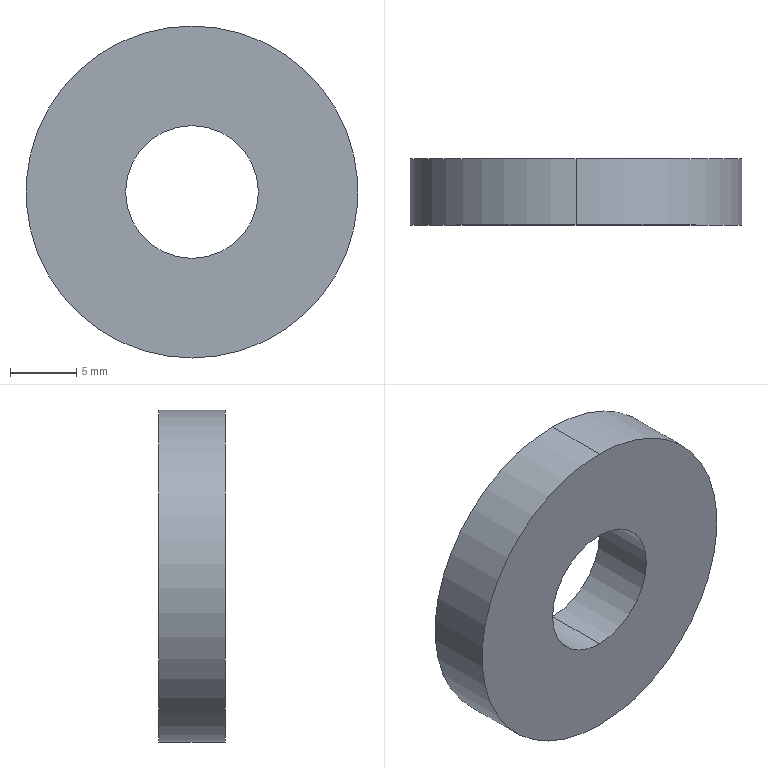Component | SolidWorks | STB-08-022-1 | 1 solid | 6 faces | box 25 x 5 x 25 mm | volume 2062 mm3 | cylinder 4 | plane 2 | commonest cylinder face diameters 10 x2 25 x2
build123d program:
from build123d import *

# Parameters (mm, degrees)
SKETCH1_R           = 12.5
BOSS_EXTRUDE1_DEPTH = 2.5
CUT_EXTRUDE1_REACH  = 20.371
SKETCH2_R           = 5


with BuildPart() as part:
    # Sketch1 → Boss-Extrude1 (new, symmetric)
    with BuildSketch(Plane(origin=(0, 0, 0), x_dir=(1, 0, 0), z_dir=(0, 1, 0))):
        with Locations(Location((0, 0, 0), (0, 0, 270))):
            Circle(SKETCH1_R)
    extrude(amount=BOSS_EXTRUDE1_DEPTH, both=True)

    # Sketch2 → Cut-Extrude1 (cut, up to next)
    with BuildSketch(Plane(origin=(0, 2.5, 0), x_dir=(1, 0, 0), z_dir=(0, 1, 0)), mode=Mode.PRIVATE) as cut_extrude1_sk1:
        with Locations(Location((0, 0, 0), (0, 0, 270))):
            Circle(SKETCH2_R)
    cut_extrude1_tool1 = extrude(cut_extrude1_sk1.sketch, amount=-CUT_EXTRUDE1_REACH, mode=Mode.PRIVATE) & part.part
    add(cut_extrude1_tool1.solids().sort_by_distance((0, 2.5, 0))[0], mode=Mode.SUBTRACT)


solid = part.part

# Placed as in the assembly
solid = solid.moved(Location((-149.904, 246.499, -12), (0, 0, 0)))
STEP:
#1=COLOUR_RGB('',0.7922,0.8196,0.9333);
#2=FILL_AREA_STYLE_COLOUR('',#1);
#3=FILL_AREA_STYLE('',(#2));
#4=SURFACE_STYLE_FILL_AREA(#3);
#5=SURFACE_SIDE_STYLE('',(#4));
#6=SURFACE_STYLE_USAGE(.BOTH.,#5);
#7=PRESENTATION_STYLE_ASSIGNMENT((#6));
#8=CARTESIAN_POINT('',(-5.902,9.606,-0.2756));
#9=VERTEX_POINT('',#8);
#10=CARTESIAN_POINT('',(-5.902,9.606,-0.6693));
#11=VERTEX_POINT('',#10);
#12=CARTESIAN_POINT('',(-5.902,9.606,-0.4724));
#13=DIRECTION('',(0.,-1.,0.));
#14=DIRECTION('',(0.,0.,1.));
#15=AXIS2_PLACEMENT_3D('',#12,#13,#14);
#16=CIRCLE('',#15,0.1969);
#17=EDGE_CURVE('',#9,#11,#16,.T.);
#18=ORIENTED_EDGE('',*,*,#17,.T.);
#19=CARTESIAN_POINT('',(-5.902,9.803,-0.6693));
#20=VERTEX_POINT('',#19);
#21=CARTESIAN_POINT('',(-5.902,9.606,-0.6693));
#22=DIRECTION('',(0.,1.,0.));
#23=VECTOR('',#22,39.37);
#24=LINE('',#21,#23);
#25=EDGE_CURVE('',#11,#20,#24,.T.);
#26=ORIENTED_EDGE('',*,*,#25,.T.);
#27=CARTESIAN_POINT('',(-5.902,9.803,-0.2756));
#28=VERTEX_POINT('',#27);
#29=CARTESIAN_POINT('',(-5.902,9.803,-0.4724));
#30=DIRECTION('',(0.,1.,0.));
#31=DIRECTION('',(0.,0.,1.));
#32=AXIS2_PLACEMENT_3D('',#29,#30,#31);
#33=CIRCLE('',#32,0.1969);
#34=EDGE_CURVE('',#20,#28,#33,.T.);
#35=ORIENTED_EDGE('',*,*,#34,.T.);
#36=CARTESIAN_POINT('',(-5.902,9.606,-0.2756));
#37=DIRECTION('',(0.,1.,0.));
#38=VECTOR('',#37,39.37);
#39=LINE('',#36,#38);
#40=EDGE_CURVE('',#9,#28,#39,.T.);
#41=ORIENTED_EDGE('',*,*,#40,.F.);
#42=EDGE_LOOP('',(#18,#26,#35,#41));
#43=FACE_OUTER_BOUND('',#42,.T.);
#44=CARTESIAN_POINT('',(-5.902,9.606,-0.4724));
#45=DIRECTION('',(0.,1.,0.));
#46=DIRECTION('',(0.,0.,1.));
#47=AXIS2_PLACEMENT_3D('',#44,#45,#46);
#48=CYLINDRICAL_SURFACE('',#47,0.1969);
#49=ADVANCED_FACE('',(#43),#48,.F.);
#50=CARTESIAN_POINT('',(-5.902,9.803,0.01969));
#51=VERTEX_POINT('',#50);
#52=CARTESIAN_POINT('',(-5.902,9.803,-0.9646));
#53=VERTEX_POINT('',#52);
#54=CARTESIAN_POINT('',(-5.902,9.803,-0.4724));
#55=DIRECTION('',(0.,1.,0.));
#56=DIRECTION('',(0.,0.,1.));
#57=AXIS2_PLACEMENT_3D('',#54,#55,#56);
#58=CIRCLE('',#57,0.4921);
#59=EDGE_CURVE('',#51,#53,#58,.T.);
#60=ORIENTED_EDGE('',*,*,#59,.F.);
#61=CARTESIAN_POINT('',(-5.902,9.606,0.01969));
#62=VERTEX_POINT('',#61);
#63=CARTESIAN_POINT('',(-5.902,9.803,0.01969));
#64=DIRECTION('',(0.,-1.,0.));
#65=VECTOR('',#64,39.37);
#66=LINE('',#63,#65);
#67=EDGE_CURVE('',#51,#62,#66,.T.);
#68=ORIENTED_EDGE('',*,*,#67,.T.);
#69=CARTESIAN_POINT('',(-5.902,9.606,-0.9646));
#70=VERTEX_POINT('',#69);
#71=CARTESIAN_POINT('',(-5.902,9.606,-0.4724));
#72=DIRECTION('',(0.,1.,0.));
#73=DIRECTION('',(0.,0.,1.));
#74=AXIS2_PLACEMENT_3D('',#71,#72,#73);
#75=CIRCLE('',#74,0.4921);
#76=EDGE_CURVE('',#62,#70,#75,.T.);
#77=ORIENTED_EDGE('',*,*,#76,.T.);
#78=CARTESIAN_POINT('',(-5.902,9.803,-0.9646));
#79=DIRECTION('',(0.,-1.,0.));
#80=VECTOR('',#79,39.37);
#81=LINE('',#78,#80);
#82=EDGE_CURVE('',#53,#70,#81,.T.);
#83=ORIENTED_EDGE('',*,*,#82,.F.);
#84=EDGE_LOOP('',(#60,#68,#77,#83));
#85=FACE_OUTER_BOUND('',#84,.T.);
#86=CARTESIAN_POINT('',(-5.902,9.803,-0.4724));
#87=DIRECTION('',(0.,-1.,0.));
#88=DIRECTION('',(0.,0.,-1.));
#89=AXIS2_PLACEMENT_3D('',#86,#87,#88);
#90=CYLINDRICAL_SURFACE('',#89,0.4921);
#91=ADVANCED_FACE('',(#85),#90,.T.);
#92=ORIENTED_EDGE('',*,*,#67,.F.);
#93=CARTESIAN_POINT('',(-5.902,9.803,-0.4724));
#94=DIRECTION('',(0.,1.,0.));
#95=DIRECTION('',(0.,0.,1.));
#96=AXIS2_PLACEMENT_3D('',#93,#94,#95);
#97=CIRCLE('',#96,0.4921);
#98=EDGE_CURVE('',#53,#51,#97,.T.);
#99=ORIENTED_EDGE('',*,*,#98,.F.);
#100=ORIENTED_EDGE('',*,*,#82,.T.);
#101=CARTESIAN_POINT('',(-5.902,9.606,-0.4724));
#102=DIRECTION('',(0.,1.,0.));
#103=DIRECTION('',(0.,0.,1.));
#104=AXIS2_PLACEMENT_3D('',#101,#102,#103);
#105=CIRCLE('',#104,0.4921);
#106=EDGE_CURVE('',#70,#62,#105,.T.);
#107=ORIENTED_EDGE('',*,*,#106,.T.);
#108=EDGE_LOOP('',(#92,#99,#100,#107));
#109=FACE_OUTER_BOUND('',#108,.T.);
#110=CARTESIAN_POINT('',(-5.902,9.803,-0.4724));
#111=DIRECTION('',(0.,-1.,0.));
#112=DIRECTION('',(0.,0.,-1.));
#113=AXIS2_PLACEMENT_3D('',#110,#111,#112);
#114=CYLINDRICAL_SURFACE('',#113,0.4921);
#115=ADVANCED_FACE('',(#109),#114,.T.);
#116=CARTESIAN_POINT('',(-5.902,9.803,-0.4724));
#117=DIRECTION('',(0.,1.,0.));
#118=DIRECTION('',(0.,0.,1.));
#119=AXIS2_PLACEMENT_3D('',#116,#117,#118);
#120=CIRCLE('',#119,0.1969);
#121=EDGE_CURVE('',#28,#20,#120,.T.);
#122=ORIENTED_EDGE('',*,*,#121,.F.);
#123=ORIENTED_EDGE('',*,*,#34,.F.);
#124=EDGE_LOOP('',(#122,#123));
#125=FACE_BOUND('',#124,.T.);
#126=ORIENTED_EDGE('',*,*,#98,.T.);
#127=ORIENTED_EDGE('',*,*,#59,.T.);
#128=EDGE_LOOP('',(#126,#127));
#129=FACE_OUTER_BOUND('',#128,.T.);
#130=CARTESIAN_POINT('',(-5.902,9.803,-0.4724));
#131=DIRECTION('',(0.,1.,0.));
#132=DIRECTION('',(0.,0.,1.));
#133=AXIS2_PLACEMENT_3D('',#130,#131,#132);
#134=PLANE('',#133);
#135=ADVANCED_FACE('',(#125,#129),#134,.T.);
#136=ORIENTED_EDGE('',*,*,#17,.F.);
#137=CARTESIAN_POINT('',(-5.902,9.606,-0.4724));
#138=DIRECTION('',(0.,-1.,0.));
#139=DIRECTION('',(0.,0.,1.));
#140=AXIS2_PLACEMENT_3D('',#137,#138,#139);
#141=CIRCLE('',#140,0.1969);
#142=EDGE_CURVE('',#11,#9,#141,.T.);
#143=ORIENTED_EDGE('',*,*,#142,.F.);
#144=EDGE_LOOP('',(#136,#143));
#145=FACE_BOUND('',#144,.T.);
#146=ORIENTED_EDGE('',*,*,#106,.F.);
#147=ORIENTED_EDGE('',*,*,#76,.F.);
#148=EDGE_LOOP('',(#146,#147));
#149=FACE_OUTER_BOUND('',#148,.T.);
#150=CARTESIAN_POINT('',(-5.902,9.606,-0.4724));
#151=DIRECTION('',(0.,1.,0.));
#152=DIRECTION('',(0.,0.,1.));
#153=AXIS2_PLACEMENT_3D('',#150,#151,#152);
#154=PLANE('',#153);
#155=ADVANCED_FACE('',(#145,#149),#154,.F.);
#156=ORIENTED_EDGE('',*,*,#25,.F.);
#157=ORIENTED_EDGE('',*,*,#142,.T.);
#158=ORIENTED_EDGE('',*,*,#40,.T.);
#159=ORIENTED_EDGE('',*,*,#121,.T.);
#160=EDGE_LOOP('',(#156,#157,#158,#159));
#161=FACE_OUTER_BOUND('',#160,.T.);
#162=CARTESIAN_POINT('',(-5.902,9.606,-0.4724));
#163=DIRECTION('',(0.,1.,0.));
#164=DIRECTION('',(0.,0.,1.));
#165=AXIS2_PLACEMENT_3D('',#162,#163,#164);
#166=CYLINDRICAL_SURFACE('',#165,0.1969);
#167=ADVANCED_FACE('',(#161),#166,.F.);
#168=CLOSED_SHELL('',(#49,#91,#115,#135,#155,#167));
#169=MANIFOLD_SOLID_BREP('',#168);
#170=STYLED_ITEM('',(#7),#169);
#171=(LENGTH_UNIT()NAMED_UNIT(*)SI_UNIT($,.METRE.));
#172=LENGTH_MEASURE_WITH_UNIT(LENGTH_MEASURE(0.0254),#171);
#173=DIMENSIONAL_EXPONENTS(1.,0.,0.,0.,0.,0.,0.);
#174=(CONVERSION_BASED_UNIT('',#172)LENGTH_UNIT()NAMED_UNIT(#173));
#175=UNCERTAINTY_MEASURE_WITH_UNIT(LENGTH_MEASURE(0.00001),#174,'','');
#176=(NAMED_UNIT(*)PLANE_ANGLE_UNIT()SI_UNIT($,.RADIAN.));
#177=(NAMED_UNIT(*)SI_UNIT($,.STERADIAN.)SOLID_ANGLE_UNIT());
#178=(GEOMETRIC_REPRESENTATION_CONTEXT(3)GLOBAL_UNCERTAINTY_ASSIGNED_CONTEXT((#175))GLOBAL_UNIT_ASSIGNED_CONTEXT((#174,#176,#177))REPRESENTATION_CONTEXT('',''));
#179=MECHANICAL_DESIGN_GEOMETRIC_PRESENTATION_REPRESENTATION('',(#170),#178);
#180=CARTESIAN_POINT('',(0.,0.,0.));
#181=DIRECTION('',(0.,0.,1.));
#182=DIRECTION('',(1.,0.,0.));
#183=AXIS2_PLACEMENT_3D('',#180,#181,#182);
#184=(LENGTH_UNIT()NAMED_UNIT(*)SI_UNIT($,.METRE.));
#185=LENGTH_MEASURE_WITH_UNIT(LENGTH_MEASURE(0.0254),#184);
#186=DIMENSIONAL_EXPONENTS(1.,0.,0.,0.,0.,0.,0.);
#187=(CONVERSION_BASED_UNIT('',#185)LENGTH_UNIT()NAMED_UNIT(#186));
#188=UNCERTAINTY_MEASURE_WITH_UNIT(LENGTH_MEASURE(0.00001),#187,'','');
#189=(NAMED_UNIT(*)PLANE_ANGLE_UNIT()SI_UNIT($,.RADIAN.));
#190=(NAMED_UNIT(*)SI_UNIT($,.STERADIAN.)SOLID_ANGLE_UNIT());
#191=(GEOMETRIC_REPRESENTATION_CONTEXT(3)GLOBAL_UNCERTAINTY_ASSIGNED_CONTEXT((#188))GLOBAL_UNIT_ASSIGNED_CONTEXT((#187,#189,#190))REPRESENTATION_CONTEXT('',''));
#192=ADVANCED_BREP_SHAPE_REPRESENTATION('',(#169,#183),#191);
#193=PRESENTATION_LAYER_ASSIGNMENT('','',(#170));